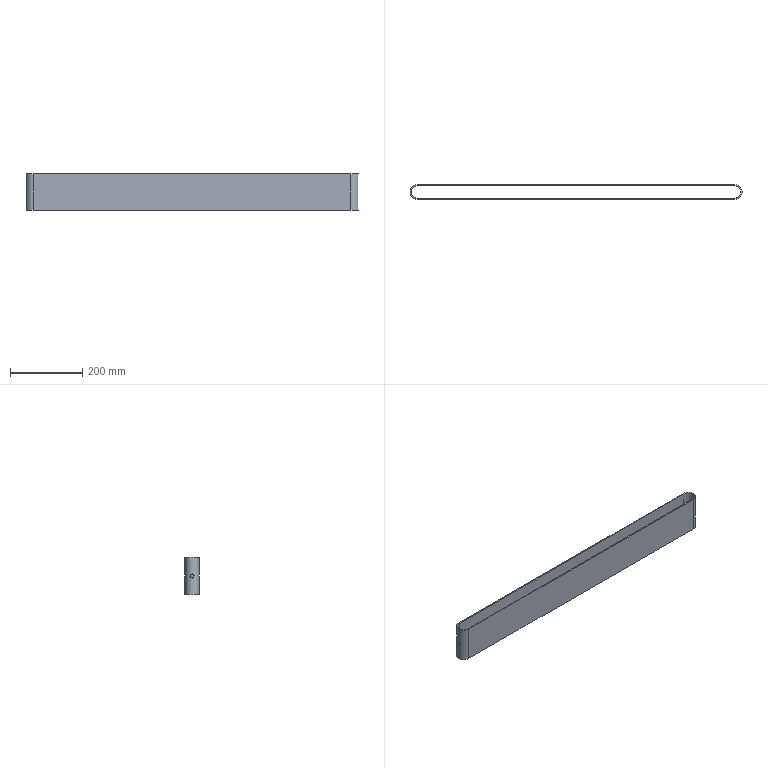Component | SolidWorks | Track-1 | 1 solid | 12 faces | box 920 x 40 x 100 mm | volume 562573 mm3 | cylinder 6 | plane 6 | commonest cylinder face diameters 11.2 x2 40 x2 34 x2
build123d program:
from build123d import *

# Parameters (mm, degrees)
BOSS_EXTRUDE1_DEPTH = 100
SKETCH2_R           = 5.6
CUT_EXTRUDE1_DEPTH  = 630.75


with BuildPart() as part:
    # Sketch1 → Boss-Extrude1 (new body)
    with BuildSketch(Plane.XY):
        with BuildLine():
            Line((91.434, 285), (91.434, -595))
            ThreePointArc((91.434, -595), (71.434, -615), (51.434, -595))
            Line((51.434, -595), (51.434, 285))
            ThreePointArc((51.434, 285), (71.434, 305), (91.434, 285))
        make_face()
        with BuildLine():
            Line((88.434, 285), (88.434, -595))
            ThreePointArc((88.434, -595), (71.434, -612), (54.434, -595))
            Line((54.434, -595), (54.434, 285))
            ThreePointArc((54.434, 285), (71.434, 302), (88.434, 285))
        make_face(mode=Mode.SUBTRACT)
    extrude(amount=BOSS_EXTRUDE1_DEPTH)

    # Sketch2 → Cut-Extrude1 (cut, through all)
    with BuildSketch(Plane(origin=(0, 0, 0), x_dir=(1, 0, 0), z_dir=(0, 1, 0))):
        with Locations(Location((71.434, -50, 0), (0, 0, 90))):
            Circle(SKETCH2_R)
    extrude(amount=CUT_EXTRUDE1_DEPTH, mode=Mode.SUBTRACT)


solid = part.part

# Placed as in the assembly
solid = solid.moved(Location((-155, 20.566, -50), (0, 0, 90)))
STEP:
#1=CARTESIAN_POINT('',(-18.11,3.622,-0.2205));
#2=VERTEX_POINT('',#1);
#3=CARTESIAN_POINT('',(-18.11,3.622,0.2205));
#4=VERTEX_POINT('',#3);
#5=CARTESIAN_POINT('',(-18.11,3.622,-0.2205));
#6=CARTESIAN_POINT('',(-18.11,3.607,-0.2205));
#7=CARTESIAN_POINT('',(-18.11,3.593,-0.219));
#8=CARTESIAN_POINT('',(-18.109,3.572,-0.2148));
#9=CARTESIAN_POINT('',(-18.108,3.565,-0.213));
#10=CARTESIAN_POINT('',(-18.107,3.551,-0.2088));
#11=CARTESIAN_POINT('',(-18.106,3.544,-0.2063));
#12=CARTESIAN_POINT('',(-18.104,3.524,-0.198));
#13=CARTESIAN_POINT('',(-18.103,3.511,-0.1912));
#14=CARTESIAN_POINT('',(-18.099,3.487,-0.1752));
#15=CARTESIAN_POINT('',(-18.097,3.476,-0.166));
#16=CARTESIAN_POINT('',(-18.093,3.456,-0.1457));
#17=CARTESIAN_POINT('',(-18.091,3.447,-0.1347));
#18=CARTESIAN_POINT('',(-18.087,3.431,-0.1106));
#19=CARTESIAN_POINT('',(-18.085,3.424,-0.09788));
#20=CARTESIAN_POINT('',(-18.083,3.416,-0.07801));
#21=CARTESIAN_POINT('',(-18.082,3.413,-0.07124));
#22=CARTESIAN_POINT('',(-18.081,3.409,-0.0574));
#23=CARTESIAN_POINT('',(-18.08,3.407,-0.05029));
#24=CARTESIAN_POINT('',(-18.079,3.403,-0.02891));
#25=CARTESIAN_POINT('',(-18.079,3.402,-0.01456));
#26=CARTESIAN_POINT('',(-18.079,3.402,0.01436));
#27=CARTESIAN_POINT('',(-18.079,3.403,0.02906));
#28=CARTESIAN_POINT('',(-18.081,3.409,0.0574));
#29=CARTESIAN_POINT('',(-18.082,3.413,0.07118));
#30=CARTESIAN_POINT('',(-18.084,3.421,0.09127));
#31=CARTESIAN_POINT('',(-18.085,3.424,0.09785));
#32=CARTESIAN_POINT('',(-18.087,3.431,0.1105));
#33=CARTESIAN_POINT('',(-18.088,3.435,0.1167));
#34=CARTESIAN_POINT('',(-18.09,3.443,0.1286));
#35=CARTESIAN_POINT('',(-18.091,3.447,0.1343));
#36=CARTESIAN_POINT('',(-18.093,3.456,0.1455));
#37=CARTESIAN_POINT('',(-18.094,3.461,0.1508));
#38=CARTESIAN_POINT('',(-18.097,3.476,0.1661));
#39=CARTESIAN_POINT('',(-18.099,3.487,0.1752));
#40=CARTESIAN_POINT('',(-18.102,3.511,0.1912));
#41=CARTESIAN_POINT('',(-18.104,3.524,0.1981));
#42=CARTESIAN_POINT('',(-18.107,3.551,0.2091));
#43=CARTESIAN_POINT('',(-18.108,3.565,0.2133));
#44=CARTESIAN_POINT('',(-18.109,3.586,0.2176));
#45=CARTESIAN_POINT('',(-18.11,3.593,0.2187));
#46=CARTESIAN_POINT('',(-18.11,3.608,0.2201));
#47=CARTESIAN_POINT('',(-18.11,3.615,0.2205));
#48=CARTESIAN_POINT('',(-18.11,3.622,0.2205));
#49=B_SPLINE_CURVE_WITH_KNOTS('',3,(#5,#6,#7,#8,#9,#10,#11,#12,#13,#14,#15,#16,#17,#18,#19,#20,#21,#22,#23,#24,#25,#26,#27,#28,#29,#30,#31,#32,#33,#34,#35,#36,#37,#38,#39,#40,#41,#42,#43,#44,#45,#46,#47,#48),.UNSPECIFIED.,.F.,.F.,(4,2,2,2,2,2,2,2,2,2,2,2,2,2,2,2,2,2,2,2,2,4),(0.,0.0011,0.00165,0.0022,0.003299,0.004399,0.005499,0.006599,0.007149,0.007698,0.008798,0.009898,0.011,0.01155,0.0121,0.01265,0.0132,0.0143,0.0154,0.0165,0.01705,0.0176),.UNSPECIFIED.);
#50=EDGE_CURVE('',#2,#4,#49,.T.);
#51=ORIENTED_EDGE('',*,*,#50,.T.);
#52=CARTESIAN_POINT('',(-17.992,3.622,0.2205));
#53=VERTEX_POINT('',#52);
#54=CARTESIAN_POINT('',(-18.11,3.622,0.2205));
#55=DIRECTION('',(1.,0.,0.));
#56=VECTOR('',#55,39.37);
#57=LINE('',#54,#56);
#58=EDGE_CURVE('',#4,#53,#57,.T.);
#59=ORIENTED_EDGE('',*,*,#58,.T.);
#60=CARTESIAN_POINT('',(-17.992,3.622,-0.2205));
#61=VERTEX_POINT('',#60);
#62=CARTESIAN_POINT('',(-17.992,3.622,-0.2205));
#63=CARTESIAN_POINT('',(-17.992,3.607,-0.2205));
#64=CARTESIAN_POINT('',(-17.992,3.593,-0.219));
#65=CARTESIAN_POINT('',(-17.99,3.572,-0.2148));
#66=CARTESIAN_POINT('',(-17.99,3.565,-0.213));
#67=CARTESIAN_POINT('',(-17.988,3.551,-0.2088));
#68=CARTESIAN_POINT('',(-17.988,3.544,-0.2063));
#69=CARTESIAN_POINT('',(-17.985,3.524,-0.198));
#70=CARTESIAN_POINT('',(-17.983,3.511,-0.1912));
#71=CARTESIAN_POINT('',(-17.98,3.493,-0.1792));
#72=CARTESIAN_POINT('',(-17.978,3.488,-0.1748));
#73=CARTESIAN_POINT('',(-17.976,3.476,-0.1657));
#74=CARTESIAN_POINT('',(-17.975,3.471,-0.1609));
#75=CARTESIAN_POINT('',(-17.971,3.456,-0.1457));
#76=CARTESIAN_POINT('',(-17.969,3.447,-0.1347));
#77=CARTESIAN_POINT('',(-17.964,3.431,-0.1106));
#78=CARTESIAN_POINT('',(-17.962,3.424,-0.09797));
#79=CARTESIAN_POINT('',(-17.96,3.416,-0.07811));
#80=CARTESIAN_POINT('',(-17.959,3.413,-0.07134));
#81=CARTESIAN_POINT('',(-17.957,3.409,-0.05748));
#82=CARTESIAN_POINT('',(-17.957,3.407,-0.05036));
#83=CARTESIAN_POINT('',(-17.955,3.403,-0.02898));
#84=CARTESIAN_POINT('',(-17.955,3.402,-0.0146));
#85=CARTESIAN_POINT('',(-17.955,3.402,0.01439));
#86=CARTESIAN_POINT('',(-17.955,3.403,0.02911));
#87=CARTESIAN_POINT('',(-17.957,3.409,0.05748));
#88=CARTESIAN_POINT('',(-17.959,3.413,0.07128));
#89=CARTESIAN_POINT('',(-17.962,3.424,0.0981));
#90=CARTESIAN_POINT('',(-17.964,3.431,0.1108));
#91=CARTESIAN_POINT('',(-17.968,3.443,0.1286));
#92=CARTESIAN_POINT('',(-17.969,3.447,0.1344));
#93=CARTESIAN_POINT('',(-17.971,3.456,0.1455));
#94=CARTESIAN_POINT('',(-17.973,3.461,0.1509));
#95=CARTESIAN_POINT('',(-17.976,3.476,0.1661));
#96=CARTESIAN_POINT('',(-17.979,3.487,0.1752));
#97=CARTESIAN_POINT('',(-17.983,3.511,0.1911));
#98=CARTESIAN_POINT('',(-17.985,3.524,0.1981));
#99=CARTESIAN_POINT('',(-17.988,3.551,0.2091));
#100=CARTESIAN_POINT('',(-17.99,3.564,0.2133));
#101=CARTESIAN_POINT('',(-17.991,3.586,0.2176));
#102=CARTESIAN_POINT('',(-17.992,3.593,0.2187));
#103=CARTESIAN_POINT('',(-17.992,3.608,0.2201));
#104=CARTESIAN_POINT('',(-17.992,3.615,0.2205));
#105=CARTESIAN_POINT('',(-17.992,3.622,0.2205));
#106=B_SPLINE_CURVE_WITH_KNOTS('',3,(#62,#63,#64,#65,#66,#67,#68,#69,#70,#71,#72,#73,#74,#75,#76,#77,#78,#79,#80,#81,#82,#83,#84,#85,#86,#87,#88,#89,#90,#91,#92,#93,#94,#95,#96,#97,#98,#99,#100,#101,#102,#103,#104,#105),.UNSPECIFIED.,.F.,.F.,(4,2,2,2,2,2,2,2,2,2,2,2,2,2,2,2,2,2,2,2,2,4),(0.,0.001102,0.001653,0.002204,0.003306,0.003857,0.004408,0.00551,0.006612,0.007163,0.007714,0.008816,0.009918,0.01102,0.01212,0.01267,0.01322,0.01433,0.01543,0.01653,0.01708,0.01763),.UNSPECIFIED.);
#107=EDGE_CURVE('',#61,#53,#106,.T.);
#108=ORIENTED_EDGE('',*,*,#107,.F.);
#109=CARTESIAN_POINT('',(-18.11,3.622,-0.2205));
#110=DIRECTION('',(1.,0.,0.));
#111=VECTOR('',#110,39.37);
#112=LINE('',#109,#111);
#113=EDGE_CURVE('',#2,#61,#112,.T.);
#114=ORIENTED_EDGE('',*,*,#113,.F.);
#115=EDGE_LOOP('',(#51,#59,#108,#114));
#116=FACE_OUTER_BOUND('',#115,.T.);
#117=CARTESIAN_POINT('',(-18.11,3.622,0.));
#118=DIRECTION('',(1.,0.,0.));
#119=DIRECTION('',(0.,0.,-1.));
#120=AXIS2_PLACEMENT_3D('',#117,#118,#119);
#121=CYLINDRICAL_SURFACE('',#120,0.2205);
#122=ADVANCED_FACE('',(#116),#121,.F.);
#123=CARTESIAN_POINT('',(-17.323,4.409,-1.969));
#124=VERTEX_POINT('',#123);
#125=CARTESIAN_POINT('',(-17.323,2.835,-1.969));
#126=VERTEX_POINT('',#125);
#127=CARTESIAN_POINT('',(-17.323,3.622,-1.969));
#128=DIRECTION('',(0.,0.,1.));
#129=DIRECTION('',(0.,1.,0.));
#130=AXIS2_PLACEMENT_3D('',#127,#128,#129);
#131=CIRCLE('',#130,0.7874);
#132=EDGE_CURVE('',#124,#126,#131,.T.);
#133=ORIENTED_EDGE('',*,*,#132,.T.);
#134=CARTESIAN_POINT('',(-17.323,2.835,1.969));
#135=VERTEX_POINT('',#134);
#136=CARTESIAN_POINT('',(-17.323,2.835,1.969));
#137=DIRECTION('',(0.,0.,-1.));
#138=VECTOR('',#137,39.37);
#139=LINE('',#136,#138);
#140=EDGE_CURVE('',#135,#126,#139,.T.);
#141=ORIENTED_EDGE('',*,*,#140,.F.);
#142=CARTESIAN_POINT('',(-17.323,4.409,1.969));
#143=VERTEX_POINT('',#142);
#144=CARTESIAN_POINT('',(-17.323,3.622,1.969));
#145=DIRECTION('',(0.,0.,1.));
#146=DIRECTION('',(0.,1.,0.));
#147=AXIS2_PLACEMENT_3D('',#144,#145,#146);
#148=CIRCLE('',#147,0.7874);
#149=EDGE_CURVE('',#143,#135,#148,.T.);
#150=ORIENTED_EDGE('',*,*,#149,.F.);
#151=CARTESIAN_POINT('',(-17.323,4.409,1.969));
#152=DIRECTION('',(0.,0.,-1.));
#153=VECTOR('',#152,39.37);
#154=LINE('',#151,#153);
#155=EDGE_CURVE('',#143,#124,#154,.T.);
#156=ORIENTED_EDGE('',*,*,#155,.T.);
#157=EDGE_LOOP('',(#133,#141,#150,#156));
#158=FACE_OUTER_BOUND('',#157,.T.);
#159=ORIENTED_EDGE('',*,*,#50,.F.);
#160=CARTESIAN_POINT('',(-18.11,3.622,0.2205));
#161=CARTESIAN_POINT('',(-18.11,3.636,0.2205));
#162=CARTESIAN_POINT('',(-18.11,3.651,0.2191));
#163=CARTESIAN_POINT('',(-18.108,3.68,0.2133));
#164=CARTESIAN_POINT('',(-18.107,3.693,0.2091));
#165=CARTESIAN_POINT('',(-18.104,3.72,0.1981));
#166=CARTESIAN_POINT('',(-18.103,3.733,0.1912));
#167=CARTESIAN_POINT('',(-18.099,3.757,0.1752));
#168=CARTESIAN_POINT('',(-18.097,3.768,0.1661));
#169=CARTESIAN_POINT('',(-18.094,3.783,0.1509));
#170=CARTESIAN_POINT('',(-18.093,3.788,0.1455));
#171=CARTESIAN_POINT('',(-18.091,3.797,0.1343));
#172=CARTESIAN_POINT('',(-18.09,3.801,0.1286));
#173=CARTESIAN_POINT('',(-18.087,3.813,0.1107));
#174=CARTESIAN_POINT('',(-18.085,3.82,0.09811));
#175=CARTESIAN_POINT('',(-18.082,3.831,0.07124));
#176=CARTESIAN_POINT('',(-18.081,3.835,0.05742));
#177=CARTESIAN_POINT('',(-18.08,3.84,0.03625));
#178=CARTESIAN_POINT('',(-18.079,3.841,0.0291));
#179=CARTESIAN_POINT('',(-18.079,3.842,0.01465));
#180=CARTESIAN_POINT('',(-18.079,3.843,0.007307));
#181=CARTESIAN_POINT('',(-18.079,3.843,-0.0145));
#182=CARTESIAN_POINT('',(-18.079,3.841,-0.02885));
#183=CARTESIAN_POINT('',(-18.081,3.835,-0.05722));
#184=CARTESIAN_POINT('',(-18.082,3.831,-0.07129));
#185=CARTESIAN_POINT('',(-18.085,3.82,-0.09786));
#186=CARTESIAN_POINT('',(-18.087,3.813,-0.1105));
#187=CARTESIAN_POINT('',(-18.091,3.797,-0.1346));
#188=CARTESIAN_POINT('',(-18.093,3.788,-0.1457));
#189=CARTESIAN_POINT('',(-18.096,3.773,-0.1609));
#190=CARTESIAN_POINT('',(-18.097,3.768,-0.1657));
#191=CARTESIAN_POINT('',(-18.099,3.757,-0.1748));
#192=CARTESIAN_POINT('',(-18.1,3.751,-0.1792));
#193=CARTESIAN_POINT('',(-18.103,3.733,-0.1912));
#194=CARTESIAN_POINT('',(-18.104,3.72,-0.198));
#195=CARTESIAN_POINT('',(-18.107,3.694,-0.209));
#196=CARTESIAN_POINT('',(-18.108,3.679,-0.2134));
#197=CARTESIAN_POINT('',(-18.11,3.651,-0.219));
#198=CARTESIAN_POINT('',(-18.11,3.637,-0.2205));
#199=CARTESIAN_POINT('',(-18.11,3.622,-0.2205));
#200=B_SPLINE_CURVE_WITH_KNOTS('',3,(#160,#161,#162,#163,#164,#165,#166,#167,#168,#169,#170,#171,#172,#173,#174,#175,#176,#177,#178,#179,#180,#181,#182,#183,#184,#185,#186,#187,#188,#189,#190,#191,#192,#193,#194,#195,#196,#197,#198,#199),.UNSPECIFIED.,.F.,.F.,(4,2,2,2,2,2,2,2,2,2,2,2,2,2,2,2,2,2,2,4),(0.0176,0.0187,0.0198,0.02089,0.02199,0.02254,0.02309,0.02419,0.02529,0.02584,0.02639,0.02749,0.02859,0.02969,0.03079,0.03134,0.03189,0.03299,0.03409,0.03519),.UNSPECIFIED.);
#201=EDGE_CURVE('',#4,#2,#200,.T.);
#202=ORIENTED_EDGE('',*,*,#201,.F.);
#203=EDGE_LOOP('',(#159,#202));
#204=FACE_BOUND('',#203,.T.);
#205=CARTESIAN_POINT('',(-17.323,3.622,1.969));
#206=DIRECTION('',(0.,0.,-1.));
#207=DIRECTION('',(0.,-1.,0.));
#208=AXIS2_PLACEMENT_3D('',#205,#206,#207);
#209=CYLINDRICAL_SURFACE('',#208,0.7874);
#210=ADVANCED_FACE('',(#158,#204),#209,.T.);
#211=CARTESIAN_POINT('',(-17.323,4.291,-1.969));
#212=VERTEX_POINT('',#211);
#213=CARTESIAN_POINT('',(-17.323,2.953,-1.969));
#214=VERTEX_POINT('',#213);
#215=CARTESIAN_POINT('',(-17.323,3.622,-1.969));
#216=DIRECTION('',(0.,0.,1.));
#217=DIRECTION('',(0.,1.,0.));
#218=AXIS2_PLACEMENT_3D('',#215,#216,#217);
#219=CIRCLE('',#218,0.6693);
#220=EDGE_CURVE('',#212,#214,#219,.T.);
#221=ORIENTED_EDGE('',*,*,#220,.F.);
#222=CARTESIAN_POINT('',(-17.323,4.291,1.969));
#223=VERTEX_POINT('',#222);
#224=CARTESIAN_POINT('',(-17.323,4.291,1.969));
#225=DIRECTION('',(0.,0.,-1.));
#226=VECTOR('',#225,39.37);
#227=LINE('',#224,#226);
#228=EDGE_CURVE('',#223,#212,#227,.T.);
#229=ORIENTED_EDGE('',*,*,#228,.F.);
#230=CARTESIAN_POINT('',(-17.323,2.953,1.969));
#231=VERTEX_POINT('',#230);
#232=CARTESIAN_POINT('',(-17.323,3.622,1.969));
#233=DIRECTION('',(0.,0.,1.));
#234=DIRECTION('',(0.,1.,0.));
#235=AXIS2_PLACEMENT_3D('',#232,#233,#234);
#236=CIRCLE('',#235,0.6693);
#237=EDGE_CURVE('',#223,#231,#236,.T.);
#238=ORIENTED_EDGE('',*,*,#237,.T.);
#239=CARTESIAN_POINT('',(-17.323,2.953,1.969));
#240=DIRECTION('',(0.,0.,-1.));
#241=VECTOR('',#240,39.37);
#242=LINE('',#239,#241);
#243=EDGE_CURVE('',#231,#214,#242,.T.);
#244=ORIENTED_EDGE('',*,*,#243,.T.);
#245=EDGE_LOOP('',(#221,#229,#238,#244));
#246=FACE_OUTER_BOUND('',#245,.T.);
#247=ORIENTED_EDGE('',*,*,#107,.T.);
#248=CARTESIAN_POINT('',(-17.992,3.622,0.2205));
#249=CARTESIAN_POINT('',(-17.992,3.629,0.2205));
#250=CARTESIAN_POINT('',(-17.992,3.636,0.2201));
#251=CARTESIAN_POINT('',(-17.992,3.651,0.2187));
#252=CARTESIAN_POINT('',(-17.991,3.658,0.2176));
#253=CARTESIAN_POINT('',(-17.99,3.68,0.2133));
#254=CARTESIAN_POINT('',(-17.988,3.693,0.2091));
#255=CARTESIAN_POINT('',(-17.985,3.72,0.198));
#256=CARTESIAN_POINT('',(-17.983,3.733,0.1911));
#257=CARTESIAN_POINT('',(-17.979,3.757,0.1751));
#258=CARTESIAN_POINT('',(-17.976,3.768,0.1661));
#259=CARTESIAN_POINT('',(-17.972,3.783,0.1508));
#260=CARTESIAN_POINT('',(-17.971,3.788,0.1454));
#261=CARTESIAN_POINT('',(-17.969,3.797,0.1343));
#262=CARTESIAN_POINT('',(-17.968,3.801,0.1286));
#263=CARTESIAN_POINT('',(-17.964,3.813,0.1108));
#264=CARTESIAN_POINT('',(-17.962,3.82,0.09807));
#265=CARTESIAN_POINT('',(-17.959,3.831,0.07127));
#266=CARTESIAN_POINT('',(-17.957,3.835,0.0575));
#267=CARTESIAN_POINT('',(-17.956,3.84,0.03628));
#268=CARTESIAN_POINT('',(-17.955,3.841,0.02912));
#269=CARTESIAN_POINT('',(-17.955,3.842,0.01459));
#270=CARTESIAN_POINT('',(-17.955,3.843,0.007243));
#271=CARTESIAN_POINT('',(-17.955,3.843,-0.01455));
#272=CARTESIAN_POINT('',(-17.955,3.841,-0.02893));
#273=CARTESIAN_POINT('',(-17.957,3.837,-0.05029));
#274=CARTESIAN_POINT('',(-17.957,3.835,-0.05741));
#275=CARTESIAN_POINT('',(-17.959,3.831,-0.0713));
#276=CARTESIAN_POINT('',(-17.96,3.828,-0.07808));
#277=CARTESIAN_POINT('',(-17.962,3.82,-0.09799));
#278=CARTESIAN_POINT('',(-17.964,3.813,-0.1107));
#279=CARTESIAN_POINT('',(-17.969,3.797,-0.1347));
#280=CARTESIAN_POINT('',(-17.971,3.788,-0.1458));
#281=CARTESIAN_POINT('',(-17.976,3.768,-0.166));
#282=CARTESIAN_POINT('',(-17.979,3.757,-0.1752));
#283=CARTESIAN_POINT('',(-17.983,3.733,-0.1912));
#284=CARTESIAN_POINT('',(-17.985,3.72,-0.198));
#285=CARTESIAN_POINT('',(-17.988,3.7,-0.2063));
#286=CARTESIAN_POINT('',(-17.988,3.693,-0.2088));
#287=CARTESIAN_POINT('',(-17.99,3.679,-0.213));
#288=CARTESIAN_POINT('',(-17.99,3.672,-0.2148));
#289=CARTESIAN_POINT('',(-17.992,3.651,-0.219));
#290=CARTESIAN_POINT('',(-17.992,3.637,-0.2205));
#291=CARTESIAN_POINT('',(-17.992,3.622,-0.2205));
#292=B_SPLINE_CURVE_WITH_KNOTS('',3,(#248,#249,#250,#251,#252,#253,#254,#255,#256,#257,#258,#259,#260,#261,#262,#263,#264,#265,#266,#267,#268,#269,#270,#271,#272,#273,#274,#275,#276,#277,#278,#279,#280,#281,#282,#283,#284,#285,#286,#287,#288,#289,#290,#291),.UNSPECIFIED.,.F.,.F.,(4,2,2,2,2,2,2,2,2,2,2,2,2,2,2,2,2,2,2,2,2,4),(0.01763,0.01818,0.01873,0.01984,0.02094,0.02204,0.02259,0.02314,0.02424,0.02534,0.0259,0.02645,0.02755,0.0281,0.02865,0.02975,0.03085,0.03195,0.03306,0.03361,0.03416,0.03526),.UNSPECIFIED.);
#293=EDGE_CURVE('',#53,#61,#292,.T.);
#294=ORIENTED_EDGE('',*,*,#293,.T.);
#295=EDGE_LOOP('',(#247,#294));
#296=FACE_BOUND('',#295,.T.);
#297=CARTESIAN_POINT('',(-17.323,3.622,1.969));
#298=DIRECTION('',(0.,0.,-1.));
#299=DIRECTION('',(0.,-1.,0.));
#300=AXIS2_PLACEMENT_3D('',#297,#298,#299);
#301=CYLINDRICAL_SURFACE('',#300,0.6693);
#302=ADVANCED_FACE('',(#246,#296),#301,.F.);
#303=ORIENTED_EDGE('',*,*,#149,.T.);
#304=CARTESIAN_POINT('',(17.323,2.835,1.969));
#305=VERTEX_POINT('',#304);
#306=CARTESIAN_POINT('',(-17.323,2.835,1.969));
#307=DIRECTION('',(1.,-0.,0.));
#308=VECTOR('',#307,39.37);
#309=LINE('',#306,#308);
#310=EDGE_CURVE('',#135,#305,#309,.T.);
#311=ORIENTED_EDGE('',*,*,#310,.T.);
#312=CARTESIAN_POINT('',(17.323,4.409,1.969));
#313=VERTEX_POINT('',#312);
#314=CARTESIAN_POINT('',(17.323,3.622,1.969));
#315=DIRECTION('',(0.,0.,1.));
#316=DIRECTION('',(0.,1.,0.));
#317=AXIS2_PLACEMENT_3D('',#314,#315,#316);
#318=CIRCLE('',#317,0.7874);
#319=EDGE_CURVE('',#305,#313,#318,.T.);
#320=ORIENTED_EDGE('',*,*,#319,.T.);
#321=CARTESIAN_POINT('',(-17.323,4.409,1.969));
#322=DIRECTION('',(-1.,0.,0.));
#323=VECTOR('',#322,39.37);
#324=LINE('',#321,#323);
#325=EDGE_CURVE('',#313,#143,#324,.T.);
#326=ORIENTED_EDGE('',*,*,#325,.T.);
#327=EDGE_LOOP('',(#303,#311,#320,#326));
#328=FACE_OUTER_BOUND('',#327,.T.);
#329=CARTESIAN_POINT('',(17.323,2.953,1.969));
#330=VERTEX_POINT('',#329);
#331=CARTESIAN_POINT('',(-17.323,2.953,1.969));
#332=DIRECTION('',(1.,-0.,0.));
#333=VECTOR('',#332,39.37);
#334=LINE('',#331,#333);
#335=EDGE_CURVE('',#231,#330,#334,.T.);
#336=ORIENTED_EDGE('',*,*,#335,.F.);
#337=ORIENTED_EDGE('',*,*,#237,.F.);
#338=CARTESIAN_POINT('',(17.323,4.291,1.969));
#339=VERTEX_POINT('',#338);
#340=CARTESIAN_POINT('',(-17.323,4.291,1.969));
#341=DIRECTION('',(-1.,0.,0.));
#342=VECTOR('',#341,39.37);
#343=LINE('',#340,#342);
#344=EDGE_CURVE('',#339,#223,#343,.T.);
#345=ORIENTED_EDGE('',*,*,#344,.F.);
#346=CARTESIAN_POINT('',(17.323,3.622,1.969));
#347=DIRECTION('',(0.,0.,1.));
#348=DIRECTION('',(0.,1.,0.));
#349=AXIS2_PLACEMENT_3D('',#346,#347,#348);
#350=CIRCLE('',#349,0.6693);
#351=EDGE_CURVE('',#330,#339,#350,.T.);
#352=ORIENTED_EDGE('',*,*,#351,.F.);
#353=EDGE_LOOP('',(#336,#337,#345,#352));
#354=FACE_BOUND('',#353,.T.);
#355=CARTESIAN_POINT('',(-17.323,3.622,1.969));
#356=DIRECTION('',(0.,0.,1.));
#357=DIRECTION('',(0.,1.,0.));
#358=AXIS2_PLACEMENT_3D('',#355,#356,#357);
#359=PLANE('',#358);
#360=ADVANCED_FACE('',(#328,#354),#359,.T.);
#361=ORIENTED_EDGE('',*,*,#132,.F.);
#362=CARTESIAN_POINT('',(17.323,4.409,-1.969));
#363=VERTEX_POINT('',#362);
#364=CARTESIAN_POINT('',(-17.323,4.409,-1.969));
#365=DIRECTION('',(-1.,0.,0.));
#366=VECTOR('',#365,39.37);
#367=LINE('',#364,#366);
#368=EDGE_CURVE('',#363,#124,#367,.T.);
#369=ORIENTED_EDGE('',*,*,#368,.F.);
#370=CARTESIAN_POINT('',(17.323,2.835,-1.969));
#371=VERTEX_POINT('',#370);
#372=CARTESIAN_POINT('',(17.323,3.622,-1.969));
#373=DIRECTION('',(0.,0.,1.));
#374=DIRECTION('',(0.,1.,0.));
#375=AXIS2_PLACEMENT_3D('',#372,#373,#374);
#376=CIRCLE('',#375,0.7874);
#377=EDGE_CURVE('',#371,#363,#376,.T.);
#378=ORIENTED_EDGE('',*,*,#377,.F.);
#379=CARTESIAN_POINT('',(-17.323,2.835,-1.969));
#380=DIRECTION('',(1.,-0.,0.));
#381=VECTOR('',#380,39.37);
#382=LINE('',#379,#381);
#383=EDGE_CURVE('',#126,#371,#382,.T.);
#384=ORIENTED_EDGE('',*,*,#383,.F.);
#385=EDGE_LOOP('',(#361,#369,#378,#384));
#386=FACE_OUTER_BOUND('',#385,.T.);
#387=ORIENTED_EDGE('',*,*,#220,.T.);
#388=CARTESIAN_POINT('',(17.323,2.953,-1.969));
#389=VERTEX_POINT('',#388);
#390=CARTESIAN_POINT('',(-17.323,2.953,-1.969));
#391=DIRECTION('',(1.,-0.,0.));
#392=VECTOR('',#391,39.37);
#393=LINE('',#390,#392);
#394=EDGE_CURVE('',#214,#389,#393,.T.);
#395=ORIENTED_EDGE('',*,*,#394,.T.);
#396=CARTESIAN_POINT('',(17.323,4.291,-1.969));
#397=VERTEX_POINT('',#396);
#398=CARTESIAN_POINT('',(17.323,3.622,-1.969));
#399=DIRECTION('',(0.,0.,1.));
#400=DIRECTION('',(0.,1.,0.));
#401=AXIS2_PLACEMENT_3D('',#398,#399,#400);
#402=CIRCLE('',#401,0.6693);
#403=EDGE_CURVE('',#389,#397,#402,.T.);
#404=ORIENTED_EDGE('',*,*,#403,.T.);
#405=CARTESIAN_POINT('',(-17.323,4.291,-1.969));
#406=DIRECTION('',(-1.,0.,0.));
#407=VECTOR('',#406,39.37);
#408=LINE('',#405,#407);
#409=EDGE_CURVE('',#397,#212,#408,.T.);
#410=ORIENTED_EDGE('',*,*,#409,.T.);
#411=EDGE_LOOP('',(#387,#395,#404,#410));
#412=FACE_BOUND('',#411,.T.);
#413=CARTESIAN_POINT('',(-17.323,3.622,-1.969));
#414=DIRECTION('',(0.,0.,1.));
#415=DIRECTION('',(0.,1.,0.));
#416=AXIS2_PLACEMENT_3D('',#413,#414,#415);
#417=PLANE('',#416);
#418=ADVANCED_FACE('',(#386,#412),#417,.F.);
#419=ORIENTED_EDGE('',*,*,#383,.T.);
#420=CARTESIAN_POINT('',(17.323,2.835,1.969));
#421=DIRECTION('',(0.,0.,-1.));
#422=VECTOR('',#421,39.37);
#423=LINE('',#420,#422);
#424=EDGE_CURVE('',#305,#371,#423,.T.);
#425=ORIENTED_EDGE('',*,*,#424,.F.);
#426=ORIENTED_EDGE('',*,*,#310,.F.);
#427=ORIENTED_EDGE('',*,*,#140,.T.);
#428=EDGE_LOOP('',(#419,#425,#426,#427));
#429=FACE_OUTER_BOUND('',#428,.T.);
#430=CARTESIAN_POINT('',(-17.323,2.835,1.969));
#431=DIRECTION('',(0.,1.,0.));
#432=DIRECTION('',(-1.,0.,0.));
#433=AXIS2_PLACEMENT_3D('',#430,#431,#432);
#434=PLANE('',#433);
#435=ADVANCED_FACE('',(#429),#434,.F.);
#436=ORIENTED_EDGE('',*,*,#377,.T.);
#437=CARTESIAN_POINT('',(17.323,4.409,1.969));
#438=DIRECTION('',(0.,0.,-1.));
#439=VECTOR('',#438,39.37);
#440=LINE('',#437,#439);
#441=EDGE_CURVE('',#313,#363,#440,.T.);
#442=ORIENTED_EDGE('',*,*,#441,.F.);
#443=ORIENTED_EDGE('',*,*,#319,.F.);
#444=ORIENTED_EDGE('',*,*,#424,.T.);
#445=EDGE_LOOP('',(#436,#442,#443,#444));
#446=FACE_OUTER_BOUND('',#445,.T.);
#447=CARTESIAN_POINT('',(17.323,3.622,1.969));
#448=DIRECTION('',(0.,0.,-1.));
#449=DIRECTION('',(0.,-1.,0.));
#450=AXIS2_PLACEMENT_3D('',#447,#448,#449);
#451=CYLINDRICAL_SURFACE('',#450,0.7874);
#452=ADVANCED_FACE('',(#446),#451,.T.);
#453=ORIENTED_EDGE('',*,*,#368,.T.);
#454=ORIENTED_EDGE('',*,*,#155,.F.);
#455=ORIENTED_EDGE('',*,*,#325,.F.);
#456=ORIENTED_EDGE('',*,*,#441,.T.);
#457=EDGE_LOOP('',(#453,#454,#455,#456));
#458=FACE_OUTER_BOUND('',#457,.T.);
#459=CARTESIAN_POINT('',(-17.323,4.409,1.969));
#460=DIRECTION('',(-0.,-1.,0.));
#461=DIRECTION('',(1.,-0.,0.));
#462=AXIS2_PLACEMENT_3D('',#459,#460,#461);
#463=PLANE('',#462);
#464=ADVANCED_FACE('',(#458),#463,.F.);
#465=ORIENTED_EDGE('',*,*,#394,.F.);
#466=ORIENTED_EDGE('',*,*,#243,.F.);
#467=ORIENTED_EDGE('',*,*,#335,.T.);
#468=CARTESIAN_POINT('',(17.323,2.953,1.969));
#469=DIRECTION('',(0.,0.,-1.));
#470=VECTOR('',#469,39.37);
#471=LINE('',#468,#470);
#472=EDGE_CURVE('',#330,#389,#471,.T.);
#473=ORIENTED_EDGE('',*,*,#472,.T.);
#474=EDGE_LOOP('',(#465,#466,#467,#473));
#475=FACE_OUTER_BOUND('',#474,.T.);
#476=CARTESIAN_POINT('',(-17.323,2.953,1.969));
#477=DIRECTION('',(0.,1.,0.));
#478=DIRECTION('',(-1.,0.,0.));
#479=AXIS2_PLACEMENT_3D('',#476,#477,#478);
#480=PLANE('',#479);
#481=ADVANCED_FACE('',(#475),#480,.T.);
#482=ORIENTED_EDGE('',*,*,#403,.F.);
#483=ORIENTED_EDGE('',*,*,#472,.F.);
#484=ORIENTED_EDGE('',*,*,#351,.T.);
#485=CARTESIAN_POINT('',(17.323,4.291,1.969));
#486=DIRECTION('',(0.,0.,-1.));
#487=VECTOR('',#486,39.37);
#488=LINE('',#485,#487);
#489=EDGE_CURVE('',#339,#397,#488,.T.);
#490=ORIENTED_EDGE('',*,*,#489,.T.);
#491=EDGE_LOOP('',(#482,#483,#484,#490));
#492=FACE_OUTER_BOUND('',#491,.T.);
#493=CARTESIAN_POINT('',(17.323,3.622,1.969));
#494=DIRECTION('',(0.,0.,-1.));
#495=DIRECTION('',(0.,-1.,0.));
#496=AXIS2_PLACEMENT_3D('',#493,#494,#495);
#497=CYLINDRICAL_SURFACE('',#496,0.6693);
#498=ADVANCED_FACE('',(#492),#497,.F.);
#499=ORIENTED_EDGE('',*,*,#409,.F.);
#500=ORIENTED_EDGE('',*,*,#489,.F.);
#501=ORIENTED_EDGE('',*,*,#344,.T.);
#502=ORIENTED_EDGE('',*,*,#228,.T.);
#503=EDGE_LOOP('',(#499,#500,#501,#502));
#504=FACE_OUTER_BOUND('',#503,.T.);
#505=CARTESIAN_POINT('',(-17.323,4.291,1.969));
#506=DIRECTION('',(-0.,-1.,0.));
#507=DIRECTION('',(1.,-0.,0.));
#508=AXIS2_PLACEMENT_3D('',#505,#506,#507);
#509=PLANE('',#508);
#510=ADVANCED_FACE('',(#504),#509,.T.);
#511=ORIENTED_EDGE('',*,*,#58,.F.);
#512=ORIENTED_EDGE('',*,*,#201,.T.);
#513=ORIENTED_EDGE('',*,*,#113,.T.);
#514=ORIENTED_EDGE('',*,*,#293,.F.);
#515=EDGE_LOOP('',(#511,#512,#513,#514));
#516=FACE_OUTER_BOUND('',#515,.T.);
#517=CARTESIAN_POINT('',(-18.11,3.622,0.));
#518=DIRECTION('',(1.,0.,0.));
#519=DIRECTION('',(0.,0.,-1.));
#520=AXIS2_PLACEMENT_3D('',#517,#518,#519);
#521=CYLINDRICAL_SURFACE('',#520,0.2205);
#522=ADVANCED_FACE('',(#516),#521,.F.);
#523=CLOSED_SHELL('',(#122,#210,#302,#360,#418,#435,#452,#464,#481,#498,#510,#522));
#524=MANIFOLD_SOLID_BREP('',#523);
#525=CARTESIAN_POINT('',(0.,0.,0.));
#526=DIRECTION('',(0.,0.,1.));
#527=DIRECTION('',(1.,0.,0.));
#528=AXIS2_PLACEMENT_3D('',#525,#526,#527);
#529=(LENGTH_UNIT()NAMED_UNIT(*)SI_UNIT($,.METRE.));
#530=LENGTH_MEASURE_WITH_UNIT(LENGTH_MEASURE(0.0254),#529);
#531=DIMENSIONAL_EXPONENTS(1.,0.,0.,0.,0.,0.,0.);
#532=(CONVERSION_BASED_UNIT('',#530)LENGTH_UNIT()NAMED_UNIT(#531));
#533=UNCERTAINTY_MEASURE_WITH_UNIT(LENGTH_MEASURE(0.00001),#532,'','');
#534=(NAMED_UNIT(*)PLANE_ANGLE_UNIT()SI_UNIT($,.RADIAN.));
#535=(NAMED_UNIT(*)SI_UNIT($,.STERADIAN.)SOLID_ANGLE_UNIT());
#536=(GEOMETRIC_REPRESENTATION_CONTEXT(3)GLOBAL_UNCERTAINTY_ASSIGNED_CONTEXT((#533))GLOBAL_UNIT_ASSIGNED_CONTEXT((#532,#534,#535))REPRESENTATION_CONTEXT('',''));
#537=ADVANCED_BREP_SHAPE_REPRESENTATION('',(#524,#528),#536);
#538=COLOUR_RGB('',0.7922,0.8196,0.9333);
#539=FILL_AREA_STYLE_COLOUR('',#538);
#540=FILL_AREA_STYLE('',(#539));
#541=SURFACE_STYLE_FILL_AREA(#540);
#542=SURFACE_SIDE_STYLE('',(#541));
#543=SURFACE_STYLE_USAGE(.BOTH.,#542);
#544=PRESENTATION_STYLE_ASSIGNMENT((#543));
#545=STYLED_ITEM('',(#544),#524);
#546=(LENGTH_UNIT()NAMED_UNIT(*)SI_UNIT($,.METRE.));
#547=LENGTH_MEASURE_WITH_UNIT(LENGTH_MEASURE(0.0254),#546);
#548=DIMENSIONAL_EXPONENTS(1.,0.,0.,0.,0.,0.,0.);
#549=(CONVERSION_BASED_UNIT('',#547)LENGTH_UNIT()NAMED_UNIT(#548));
#550=UNCERTAINTY_MEASURE_WITH_UNIT(LENGTH_MEASURE(0.00001),#549,'','');
#551=(NAMED_UNIT(*)PLANE_ANGLE_UNIT()SI_UNIT($,.RADIAN.));
#552=(NAMED_UNIT(*)SI_UNIT($,.STERADIAN.)SOLID_ANGLE_UNIT());
#553=(GEOMETRIC_REPRESENTATION_CONTEXT(3)GLOBAL_UNCERTAINTY_ASSIGNED_CONTEXT((#550))GLOBAL_UNIT_ASSIGNED_CONTEXT((#549,#551,#552))REPRESENTATION_CONTEXT('',''));
#554=MECHANICAL_DESIGN_GEOMETRIC_PRESENTATION_REPRESENTATION('',(#545),#553);
#555=PRESENTATION_LAYER_ASSIGNMENT('','',(#545));